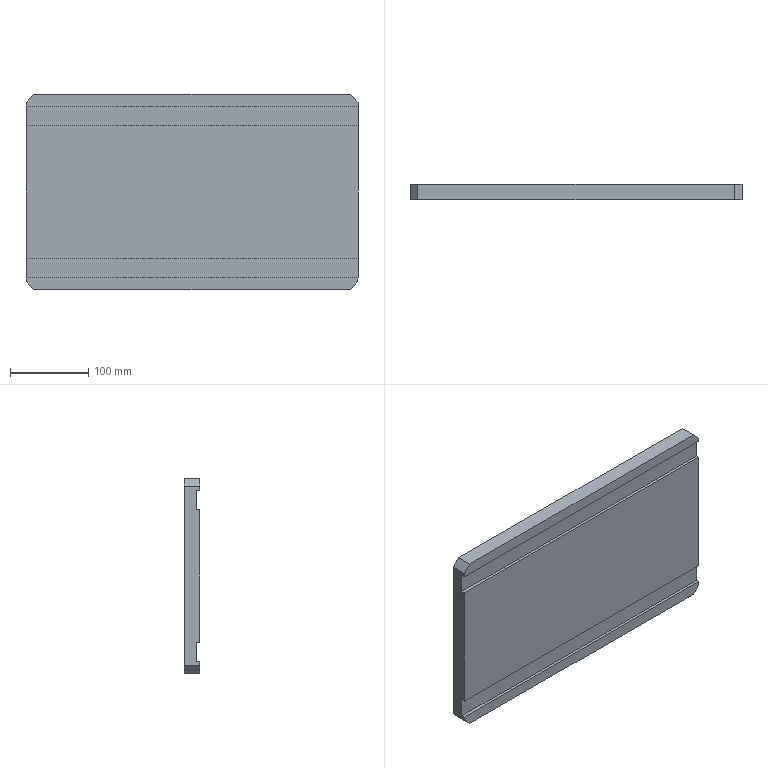Component | SolidWorks | 100-04-1 | 1 solid | 18 faces | box 425 x 20 x 250 mm | volume 2036000 mm3 | plane 18 | material 45
build123d program:
from build123d import *

# Parameters (mm, degrees)
SKETCH1_W           = 250
SKETCH1_H           = 425
BOSS_EXTRUDE1_DEPTH = 10
CHAMFER1_SIZE       = 10
SKETCH5_W           = 25
SKETCH5_H           = 425
CUT_EXTRUDE1_DEPTH  = 4


with BuildPart() as part:
    # Sketch1 → Boss-Extrude1 (new, symmetric)
    with BuildSketch(Plane(origin=(0, 0, 0), x_dir=(1, 0, 0), z_dir=(0, 1, 0))):
        Rectangle(SKETCH1_W, SKETCH1_H)
    extrude(amount=BOSS_EXTRUDE1_DEPTH, both=True)

    # Chamfer1
    chamfer1_edges = [part.edges().sort_by_distance(p)[0] for p in [
        (-125, 0, -212.5),
        (125, 0, -212.5),
        (125, 0, 212.5),
        (-125, 0, 212.5),
    ]]
    chamfer(chamfer1_edges, length=CHAMFER1_SIZE)

    # Sketch5 → Cut-Extrude1 (cut)
    with BuildSketch(Plane.XZ.offset(10)):
        with Locations((-97.5, 0)):
            Rectangle(SKETCH5_W, SKETCH5_H)
    cut_extrude1 = extrude(amount=-CUT_EXTRUDE1_DEPTH, mode=Mode.SUBTRACT)

    # Mirror1: Cut-Extrude1 across plane
    add(cut_extrude1.mirror(Plane(origin=(0, 0, 0), x_dir=(0, 0, 1), z_dir=(1, 0, 0))), mode=Mode.SUBTRACT)


solid = part.part

# Placed as in the assembly
solid = solid.moved(Location((-33.5, 990, 0), (0, 90, 0)))
STEP:
#1=COLOUR_RGB('',0.7922,0.8196,0.9333);
#2=FILL_AREA_STYLE_COLOUR('',#1);
#3=FILL_AREA_STYLE('',(#2));
#4=SURFACE_STYLE_FILL_AREA(#3);
#5=SURFACE_SIDE_STYLE('',(#4));
#6=SURFACE_STYLE_USAGE(.BOTH.,#5);
#7=PRESENTATION_STYLE_ASSIGNMENT((#6));
#8=CARTESIAN_POINT('',(7.047,38.583,3.346));
#9=VERTEX_POINT('',#8);
#10=CARTESIAN_POINT('',(-9.685,38.583,3.346));
#11=VERTEX_POINT('',#10);
#12=CARTESIAN_POINT('',(-9.685,38.583,3.346));
#13=DIRECTION('',(-1.,0.,0.));
#14=VECTOR('',#13,39.37);
#15=LINE('',#12,#14);
#16=EDGE_CURVE('',#9,#11,#15,.T.);
#17=ORIENTED_EDGE('',*,*,#16,.T.);
#18=CARTESIAN_POINT('',(-9.685,38.583,-3.346));
#19=VERTEX_POINT('',#18);
#20=CARTESIAN_POINT('',(-9.685,38.583,4.921));
#21=DIRECTION('',(0.,0.,1.));
#22=VECTOR('',#21,39.37);
#23=LINE('',#20,#22);
#24=EDGE_CURVE('',#19,#11,#23,.T.);
#25=ORIENTED_EDGE('',*,*,#24,.F.);
#26=CARTESIAN_POINT('',(7.047,38.583,-3.346));
#27=VERTEX_POINT('',#26);
#28=CARTESIAN_POINT('',(-9.685,38.583,-3.346));
#29=DIRECTION('',(-1.,0.,-0.));
#30=VECTOR('',#29,39.37);
#31=LINE('',#28,#30);
#32=EDGE_CURVE('',#27,#19,#31,.T.);
#33=ORIENTED_EDGE('',*,*,#32,.F.);
#34=CARTESIAN_POINT('',(7.047,38.583,4.921));
#35=DIRECTION('',(-0.,-0.,-1.));
#36=VECTOR('',#35,39.37);
#37=LINE('',#34,#36);
#38=EDGE_CURVE('',#9,#27,#37,.T.);
#39=ORIENTED_EDGE('',*,*,#38,.F.);
#40=EDGE_LOOP('',(#17,#25,#33,#39));
#41=FACE_OUTER_BOUND('',#40,.T.);
#42=CARTESIAN_POINT('',(-1.319,38.583,-0.));
#43=DIRECTION('',(-0.,1.,-0.));
#44=DIRECTION('',(-1.,-0.,0.));
#45=AXIS2_PLACEMENT_3D('',#42,#43,#44);
#46=PLANE('',#45);
#47=ADVANCED_FACE('',(#41),#46,.F.);
#48=CARTESIAN_POINT('',(-9.685,38.583,4.331));
#49=VERTEX_POINT('',#48);
#50=CARTESIAN_POINT('',(7.047,38.583,4.331));
#51=VERTEX_POINT('',#50);
#52=CARTESIAN_POINT('',(-9.685,38.583,4.331));
#53=DIRECTION('',(1.,-0.,-0.));
#54=VECTOR('',#53,39.37);
#55=LINE('',#52,#54);
#56=EDGE_CURVE('',#49,#51,#55,.T.);
#57=ORIENTED_EDGE('',*,*,#56,.T.);
#58=CARTESIAN_POINT('',(7.047,38.583,4.528));
#59=VERTEX_POINT('',#58);
#60=CARTESIAN_POINT('',(7.047,38.583,4.921));
#61=DIRECTION('',(-0.,-0.,-1.));
#62=VECTOR('',#61,39.37);
#63=LINE('',#60,#62);
#64=EDGE_CURVE('',#59,#51,#63,.T.);
#65=ORIENTED_EDGE('',*,*,#64,.F.);
#66=CARTESIAN_POINT('',(6.654,38.583,4.921));
#67=VERTEX_POINT('',#66);
#68=CARTESIAN_POINT('',(7.047,38.583,4.528));
#69=DIRECTION('',(-0.7071,0.,0.7071));
#70=VECTOR('',#69,39.37);
#71=LINE('',#68,#70);
#72=EDGE_CURVE('',#59,#67,#71,.T.);
#73=ORIENTED_EDGE('',*,*,#72,.T.);
#74=CARTESIAN_POINT('',(-9.291,38.583,4.921));
#75=VERTEX_POINT('',#74);
#76=CARTESIAN_POINT('',(-9.685,38.583,4.921));
#77=DIRECTION('',(1.,0.,0.));
#78=VECTOR('',#77,39.37);
#79=LINE('',#76,#78);
#80=EDGE_CURVE('',#75,#67,#79,.T.);
#81=ORIENTED_EDGE('',*,*,#80,.F.);
#82=CARTESIAN_POINT('',(-9.685,38.583,4.528));
#83=VERTEX_POINT('',#82);
#84=CARTESIAN_POINT('',(-9.291,38.583,4.921));
#85=DIRECTION('',(-0.7071,-0.,-0.7071));
#86=VECTOR('',#85,39.37);
#87=LINE('',#84,#86);
#88=EDGE_CURVE('',#75,#83,#87,.T.);
#89=ORIENTED_EDGE('',*,*,#88,.T.);
#90=CARTESIAN_POINT('',(-9.685,38.583,4.921));
#91=DIRECTION('',(0.,0.,1.));
#92=VECTOR('',#91,39.37);
#93=LINE('',#90,#92);
#94=EDGE_CURVE('',#49,#83,#93,.T.);
#95=ORIENTED_EDGE('',*,*,#94,.F.);
#96=EDGE_LOOP('',(#57,#65,#73,#81,#89,#95));
#97=FACE_OUTER_BOUND('',#96,.T.);
#98=CARTESIAN_POINT('',(-1.319,38.583,-0.));
#99=DIRECTION('',(-0.,1.,-0.));
#100=DIRECTION('',(-1.,-0.,0.));
#101=AXIS2_PLACEMENT_3D('',#98,#99,#100);
#102=PLANE('',#101);
#103=ADVANCED_FACE('',(#97),#102,.F.);
#104=CARTESIAN_POINT('',(-9.685,38.74,3.346));
#105=VERTEX_POINT('',#104);
#106=CARTESIAN_POINT('',(-9.685,38.74,3.346));
#107=DIRECTION('',(-0.,-1.,0.));
#108=VECTOR('',#107,39.37);
#109=LINE('',#106,#108);
#110=EDGE_CURVE('',#105,#11,#109,.T.);
#111=ORIENTED_EDGE('',*,*,#110,.F.);
#112=CARTESIAN_POINT('',(-9.685,38.74,4.331));
#113=VERTEX_POINT('',#112);
#114=CARTESIAN_POINT('',(-9.685,38.74,3.346));
#115=DIRECTION('',(-0.,0.,1.));
#116=VECTOR('',#115,39.37);
#117=LINE('',#114,#116);
#118=EDGE_CURVE('',#105,#113,#117,.T.);
#119=ORIENTED_EDGE('',*,*,#118,.T.);
#120=CARTESIAN_POINT('',(-9.685,38.74,4.331));
#121=DIRECTION('',(-0.,-1.,0.));
#122=VECTOR('',#121,39.37);
#123=LINE('',#120,#122);
#124=EDGE_CURVE('',#113,#49,#123,.T.);
#125=ORIENTED_EDGE('',*,*,#124,.T.);
#126=ORIENTED_EDGE('',*,*,#94,.T.);
#127=CARTESIAN_POINT('',(-9.685,39.37,4.528));
#128=VERTEX_POINT('',#127);
#129=CARTESIAN_POINT('',(-9.685,39.37,4.528));
#130=DIRECTION('',(0.,1.,-0.));
#131=VECTOR('',#130,39.37);
#132=LINE('',#129,#131);
#133=EDGE_CURVE('',#83,#128,#132,.T.);
#134=ORIENTED_EDGE('',*,*,#133,.T.);
#135=CARTESIAN_POINT('',(-9.685,39.37,-4.528));
#136=VERTEX_POINT('',#135);
#137=CARTESIAN_POINT('',(-9.685,39.37,4.921));
#138=DIRECTION('',(0.,0.,1.));
#139=VECTOR('',#138,39.37);
#140=LINE('',#137,#139);
#141=EDGE_CURVE('',#136,#128,#140,.T.);
#142=ORIENTED_EDGE('',*,*,#141,.F.);
#143=CARTESIAN_POINT('',(-9.685,38.583,-4.528));
#144=VERTEX_POINT('',#143);
#145=CARTESIAN_POINT('',(-9.685,39.37,-4.528));
#146=DIRECTION('',(-0.,-1.,0.));
#147=VECTOR('',#146,39.37);
#148=LINE('',#145,#147);
#149=EDGE_CURVE('',#136,#144,#148,.T.);
#150=ORIENTED_EDGE('',*,*,#149,.T.);
#151=CARTESIAN_POINT('',(-9.685,38.583,-4.331));
#152=VERTEX_POINT('',#151);
#153=CARTESIAN_POINT('',(-9.685,38.583,4.921));
#154=DIRECTION('',(0.,0.,1.));
#155=VECTOR('',#154,39.37);
#156=LINE('',#153,#155);
#157=EDGE_CURVE('',#144,#152,#156,.T.);
#158=ORIENTED_EDGE('',*,*,#157,.T.);
#159=CARTESIAN_POINT('',(-9.685,38.74,-4.331));
#160=VERTEX_POINT('',#159);
#161=CARTESIAN_POINT('',(-9.685,38.74,-4.331));
#162=DIRECTION('',(-0.,-1.,0.));
#163=VECTOR('',#162,39.37);
#164=LINE('',#161,#163);
#165=EDGE_CURVE('',#160,#152,#164,.T.);
#166=ORIENTED_EDGE('',*,*,#165,.F.);
#167=CARTESIAN_POINT('',(-9.685,38.74,-3.346));
#168=VERTEX_POINT('',#167);
#169=CARTESIAN_POINT('',(-9.685,38.74,-3.346));
#170=DIRECTION('',(-0.,-0.,-1.));
#171=VECTOR('',#170,39.37);
#172=LINE('',#169,#171);
#173=EDGE_CURVE('',#168,#160,#172,.T.);
#174=ORIENTED_EDGE('',*,*,#173,.F.);
#175=CARTESIAN_POINT('',(-9.685,38.74,-3.346));
#176=DIRECTION('',(-0.,-1.,0.));
#177=VECTOR('',#176,39.37);
#178=LINE('',#175,#177);
#179=EDGE_CURVE('',#168,#19,#178,.T.);
#180=ORIENTED_EDGE('',*,*,#179,.T.);
#181=ORIENTED_EDGE('',*,*,#24,.T.);
#182=EDGE_LOOP('',(#111,#119,#125,#126,#134,#142,#150,#158,#166,#174,#180,#181));
#183=FACE_OUTER_BOUND('',#182,.T.);
#184=CARTESIAN_POINT('',(-9.685,39.37,4.921));
#185=DIRECTION('',(1.,0.,-0.));
#186=DIRECTION('',(-0.,-0.,-1.));
#187=AXIS2_PLACEMENT_3D('',#184,#185,#186);
#188=PLANE('',#187);
#189=ADVANCED_FACE('',(#183),#188,.F.);
#190=CARTESIAN_POINT('',(7.047,38.74,3.346));
#191=VERTEX_POINT('',#190);
#192=CARTESIAN_POINT('',(7.047,38.74,3.346));
#193=DIRECTION('',(-0.,-1.,0.));
#194=VECTOR('',#193,39.37);
#195=LINE('',#192,#194);
#196=EDGE_CURVE('',#191,#9,#195,.T.);
#197=ORIENTED_EDGE('',*,*,#196,.T.);
#198=ORIENTED_EDGE('',*,*,#38,.T.);
#199=CARTESIAN_POINT('',(7.047,38.74,-3.346));
#200=VERTEX_POINT('',#199);
#201=CARTESIAN_POINT('',(7.047,38.74,-3.346));
#202=DIRECTION('',(-0.,-1.,0.));
#203=VECTOR('',#202,39.37);
#204=LINE('',#201,#203);
#205=EDGE_CURVE('',#200,#27,#204,.T.);
#206=ORIENTED_EDGE('',*,*,#205,.F.);
#207=CARTESIAN_POINT('',(7.047,38.74,-4.331));
#208=VERTEX_POINT('',#207);
#209=CARTESIAN_POINT('',(7.047,38.74,-3.346));
#210=DIRECTION('',(0.,0.,1.));
#211=VECTOR('',#210,39.37);
#212=LINE('',#209,#211);
#213=EDGE_CURVE('',#208,#200,#212,.T.);
#214=ORIENTED_EDGE('',*,*,#213,.F.);
#215=CARTESIAN_POINT('',(7.047,38.583,-4.331));
#216=VERTEX_POINT('',#215);
#217=CARTESIAN_POINT('',(7.047,38.74,-4.331));
#218=DIRECTION('',(-0.,-1.,0.));
#219=VECTOR('',#218,39.37);
#220=LINE('',#217,#219);
#221=EDGE_CURVE('',#208,#216,#220,.T.);
#222=ORIENTED_EDGE('',*,*,#221,.T.);
#223=CARTESIAN_POINT('',(7.047,38.583,-4.528));
#224=VERTEX_POINT('',#223);
#225=CARTESIAN_POINT('',(7.047,38.583,4.921));
#226=DIRECTION('',(-0.,-0.,-1.));
#227=VECTOR('',#226,39.37);
#228=LINE('',#225,#227);
#229=EDGE_CURVE('',#216,#224,#228,.T.);
#230=ORIENTED_EDGE('',*,*,#229,.T.);
#231=CARTESIAN_POINT('',(7.047,39.37,-4.528));
#232=VERTEX_POINT('',#231);
#233=CARTESIAN_POINT('',(7.047,39.37,-4.528));
#234=DIRECTION('',(0.,1.,-0.));
#235=VECTOR('',#234,39.37);
#236=LINE('',#233,#235);
#237=EDGE_CURVE('',#224,#232,#236,.T.);
#238=ORIENTED_EDGE('',*,*,#237,.T.);
#239=CARTESIAN_POINT('',(7.047,39.37,4.528));
#240=VERTEX_POINT('',#239);
#241=CARTESIAN_POINT('',(7.047,39.37,4.921));
#242=DIRECTION('',(-0.,-0.,-1.));
#243=VECTOR('',#242,39.37);
#244=LINE('',#241,#243);
#245=EDGE_CURVE('',#240,#232,#244,.T.);
#246=ORIENTED_EDGE('',*,*,#245,.F.);
#247=CARTESIAN_POINT('',(7.047,39.37,4.528));
#248=DIRECTION('',(-0.,-1.,0.));
#249=VECTOR('',#248,39.37);
#250=LINE('',#247,#249);
#251=EDGE_CURVE('',#240,#59,#250,.T.);
#252=ORIENTED_EDGE('',*,*,#251,.T.);
#253=ORIENTED_EDGE('',*,*,#64,.T.);
#254=CARTESIAN_POINT('',(7.047,38.74,4.331));
#255=VERTEX_POINT('',#254);
#256=CARTESIAN_POINT('',(7.047,38.74,4.331));
#257=DIRECTION('',(-0.,-1.,0.));
#258=VECTOR('',#257,39.37);
#259=LINE('',#256,#258);
#260=EDGE_CURVE('',#255,#51,#259,.T.);
#261=ORIENTED_EDGE('',*,*,#260,.F.);
#262=CARTESIAN_POINT('',(7.047,38.74,3.346));
#263=DIRECTION('',(0.,-0.,-1.));
#264=VECTOR('',#263,39.37);
#265=LINE('',#262,#264);
#266=EDGE_CURVE('',#255,#191,#265,.T.);
#267=ORIENTED_EDGE('',*,*,#266,.T.);
#268=EDGE_LOOP('',(#197,#198,#206,#214,#222,#230,#238,#246,#252,#253,#261,#267));
#269=FACE_OUTER_BOUND('',#268,.T.);
#270=CARTESIAN_POINT('',(7.047,39.37,4.921));
#271=DIRECTION('',(-1.,-0.,0.));
#272=DIRECTION('',(0.,0.,1.));
#273=AXIS2_PLACEMENT_3D('',#270,#271,#272);
#274=PLANE('',#273);
#275=ADVANCED_FACE('',(#269),#274,.F.);
#276=CARTESIAN_POINT('',(6.654,38.583,-4.921));
#277=VERTEX_POINT('',#276);
#278=CARTESIAN_POINT('',(-9.291,38.583,-4.921));
#279=VERTEX_POINT('',#278);
#280=CARTESIAN_POINT('',(-9.685,38.583,-4.921));
#281=DIRECTION('',(-1.,-0.,0.));
#282=VECTOR('',#281,39.37);
#283=LINE('',#280,#282);
#284=EDGE_CURVE('',#277,#279,#283,.T.);
#285=ORIENTED_EDGE('',*,*,#284,.T.);
#286=CARTESIAN_POINT('',(-9.291,39.37,-4.921));
#287=VERTEX_POINT('',#286);
#288=CARTESIAN_POINT('',(-9.291,39.37,-4.921));
#289=DIRECTION('',(0.,1.,-0.));
#290=VECTOR('',#289,39.37);
#291=LINE('',#288,#290);
#292=EDGE_CURVE('',#279,#287,#291,.T.);
#293=ORIENTED_EDGE('',*,*,#292,.T.);
#294=CARTESIAN_POINT('',(6.654,39.37,-4.921));
#295=VERTEX_POINT('',#294);
#296=CARTESIAN_POINT('',(-9.685,39.37,-4.921));
#297=DIRECTION('',(-1.,-0.,0.));
#298=VECTOR('',#297,39.37);
#299=LINE('',#296,#298);
#300=EDGE_CURVE('',#295,#287,#299,.T.);
#301=ORIENTED_EDGE('',*,*,#300,.F.);
#302=CARTESIAN_POINT('',(6.654,39.37,-4.921));
#303=DIRECTION('',(-0.,-1.,0.));
#304=VECTOR('',#303,39.37);
#305=LINE('',#302,#304);
#306=EDGE_CURVE('',#295,#277,#305,.T.);
#307=ORIENTED_EDGE('',*,*,#306,.T.);
#308=EDGE_LOOP('',(#285,#293,#301,#307));
#309=FACE_OUTER_BOUND('',#308,.T.);
#310=CARTESIAN_POINT('',(-9.685,39.37,-4.921));
#311=DIRECTION('',(-0.,0.,1.));
#312=DIRECTION('',(1.,0.,0.));
#313=AXIS2_PLACEMENT_3D('',#310,#311,#312);
#314=PLANE('',#313);
#315=ADVANCED_FACE('',(#309),#314,.F.);
#316=CARTESIAN_POINT('',(-9.291,39.37,4.921));
#317=VERTEX_POINT('',#316);
#318=CARTESIAN_POINT('',(6.654,39.37,4.921));
#319=VERTEX_POINT('',#318);
#320=CARTESIAN_POINT('',(-9.685,39.37,4.921));
#321=DIRECTION('',(1.,0.,0.));
#322=VECTOR('',#321,39.37);
#323=LINE('',#320,#322);
#324=EDGE_CURVE('',#317,#319,#323,.T.);
#325=ORIENTED_EDGE('',*,*,#324,.F.);
#326=CARTESIAN_POINT('',(-9.291,39.37,4.921));
#327=DIRECTION('',(-0.,-1.,0.));
#328=VECTOR('',#327,39.37);
#329=LINE('',#326,#328);
#330=EDGE_CURVE('',#317,#75,#329,.T.);
#331=ORIENTED_EDGE('',*,*,#330,.T.);
#332=ORIENTED_EDGE('',*,*,#80,.T.);
#333=CARTESIAN_POINT('',(6.654,39.37,4.921));
#334=DIRECTION('',(0.,1.,-0.));
#335=VECTOR('',#334,39.37);
#336=LINE('',#333,#335);
#337=EDGE_CURVE('',#67,#319,#336,.T.);
#338=ORIENTED_EDGE('',*,*,#337,.T.);
#339=EDGE_LOOP('',(#325,#331,#332,#338));
#340=FACE_OUTER_BOUND('',#339,.T.);
#341=CARTESIAN_POINT('',(-9.685,39.37,4.921));
#342=DIRECTION('',(0.,-0.,-1.));
#343=DIRECTION('',(-1.,-0.,0.));
#344=AXIS2_PLACEMENT_3D('',#341,#342,#343);
#345=PLANE('',#344);
#346=ADVANCED_FACE('',(#340),#345,.F.);
#347=ORIENTED_EDGE('',*,*,#300,.T.);
#348=CARTESIAN_POINT('',(-7.766,39.37,-6.447));
#349=DIRECTION('',(-0.7071,0.,0.7071));
#350=VECTOR('',#349,39.37);
#351=LINE('',#348,#350);
#352=EDGE_CURVE('',#287,#136,#351,.T.);
#353=ORIENTED_EDGE('',*,*,#352,.T.);
#354=ORIENTED_EDGE('',*,*,#141,.T.);
#355=CARTESIAN_POINT('',(-7.766,39.37,6.447));
#356=DIRECTION('',(0.7071,0.,0.7071));
#357=VECTOR('',#356,39.37);
#358=LINE('',#355,#357);
#359=EDGE_CURVE('',#128,#317,#358,.T.);
#360=ORIENTED_EDGE('',*,*,#359,.T.);
#361=ORIENTED_EDGE('',*,*,#324,.T.);
#362=CARTESIAN_POINT('',(5.128,39.37,6.447));
#363=DIRECTION('',(0.7071,-0.,-0.7071));
#364=VECTOR('',#363,39.37);
#365=LINE('',#362,#364);
#366=EDGE_CURVE('',#319,#240,#365,.T.);
#367=ORIENTED_EDGE('',*,*,#366,.T.);
#368=ORIENTED_EDGE('',*,*,#245,.T.);
#369=CARTESIAN_POINT('',(5.128,39.37,-6.447));
#370=DIRECTION('',(-0.7071,-0.,-0.7071));
#371=VECTOR('',#370,39.37);
#372=LINE('',#369,#371);
#373=EDGE_CURVE('',#232,#295,#372,.T.);
#374=ORIENTED_EDGE('',*,*,#373,.T.);
#375=EDGE_LOOP('',(#347,#353,#354,#360,#361,#367,#368,#374));
#376=FACE_OUTER_BOUND('',#375,.T.);
#377=CARTESIAN_POINT('',(-1.319,39.37,-0.));
#378=DIRECTION('',(-0.,1.,-0.));
#379=DIRECTION('',(-1.,-0.,0.));
#380=AXIS2_PLACEMENT_3D('',#377,#378,#379);
#381=PLANE('',#380);
#382=ADVANCED_FACE('',(#376),#381,.T.);
#383=ORIENTED_EDGE('',*,*,#229,.F.);
#384=CARTESIAN_POINT('',(-9.685,38.583,-4.331));
#385=DIRECTION('',(1.,-0.,0.));
#386=VECTOR('',#385,39.37);
#387=LINE('',#384,#386);
#388=EDGE_CURVE('',#152,#216,#387,.T.);
#389=ORIENTED_EDGE('',*,*,#388,.F.);
#390=ORIENTED_EDGE('',*,*,#157,.F.);
#391=CARTESIAN_POINT('',(-9.685,38.583,-4.528));
#392=DIRECTION('',(0.7071,-0.,-0.7071));
#393=VECTOR('',#392,39.37);
#394=LINE('',#391,#393);
#395=EDGE_CURVE('',#144,#279,#394,.T.);
#396=ORIENTED_EDGE('',*,*,#395,.T.);
#397=ORIENTED_EDGE('',*,*,#284,.F.);
#398=CARTESIAN_POINT('',(6.654,38.583,-4.921));
#399=DIRECTION('',(0.7071,0.,0.7071));
#400=VECTOR('',#399,39.37);
#401=LINE('',#398,#400);
#402=EDGE_CURVE('',#277,#224,#401,.T.);
#403=ORIENTED_EDGE('',*,*,#402,.T.);
#404=EDGE_LOOP('',(#383,#389,#390,#396,#397,#403));
#405=FACE_OUTER_BOUND('',#404,.T.);
#406=CARTESIAN_POINT('',(-1.319,38.583,-0.));
#407=DIRECTION('',(-0.,1.,-0.));
#408=DIRECTION('',(-1.,-0.,0.));
#409=AXIS2_PLACEMENT_3D('',#406,#407,#408);
#410=PLANE('',#409);
#411=ADVANCED_FACE('',(#405),#410,.F.);
#412=ORIENTED_EDGE('',*,*,#352,.F.);
#413=ORIENTED_EDGE('',*,*,#292,.F.);
#414=ORIENTED_EDGE('',*,*,#395,.F.);
#415=ORIENTED_EDGE('',*,*,#149,.F.);
#416=EDGE_LOOP('',(#412,#413,#414,#415));
#417=FACE_OUTER_BOUND('',#416,.T.);
#418=CARTESIAN_POINT('',(-9.685,39.37,-4.528));
#419=DIRECTION('',(0.7071,0.,0.7071));
#420=DIRECTION('',(-0.,-1.,0.));
#421=AXIS2_PLACEMENT_3D('',#418,#419,#420);
#422=PLANE('',#421);
#423=ADVANCED_FACE('',(#417),#422,.F.);
#424=ORIENTED_EDGE('',*,*,#359,.F.);
#425=ORIENTED_EDGE('',*,*,#133,.F.);
#426=ORIENTED_EDGE('',*,*,#88,.F.);
#427=ORIENTED_EDGE('',*,*,#330,.F.);
#428=EDGE_LOOP('',(#424,#425,#426,#427));
#429=FACE_OUTER_BOUND('',#428,.T.);
#430=CARTESIAN_POINT('',(-9.291,39.37,4.921));
#431=DIRECTION('',(0.7071,-0.,-0.7071));
#432=DIRECTION('',(-0.,-1.,0.));
#433=AXIS2_PLACEMENT_3D('',#430,#431,#432);
#434=PLANE('',#433);
#435=ADVANCED_FACE('',(#429),#434,.F.);
#436=ORIENTED_EDGE('',*,*,#366,.F.);
#437=ORIENTED_EDGE('',*,*,#337,.F.);
#438=ORIENTED_EDGE('',*,*,#72,.F.);
#439=ORIENTED_EDGE('',*,*,#251,.F.);
#440=EDGE_LOOP('',(#436,#437,#438,#439));
#441=FACE_OUTER_BOUND('',#440,.T.);
#442=CARTESIAN_POINT('',(7.047,39.37,4.528));
#443=DIRECTION('',(-0.7071,-0.,-0.7071));
#444=DIRECTION('',(-0.,-1.,0.));
#445=AXIS2_PLACEMENT_3D('',#442,#443,#444);
#446=PLANE('',#445);
#447=ADVANCED_FACE('',(#441),#446,.F.);
#448=ORIENTED_EDGE('',*,*,#373,.F.);
#449=ORIENTED_EDGE('',*,*,#237,.F.);
#450=ORIENTED_EDGE('',*,*,#402,.F.);
#451=ORIENTED_EDGE('',*,*,#306,.F.);
#452=EDGE_LOOP('',(#448,#449,#450,#451));
#453=FACE_OUTER_BOUND('',#452,.T.);
#454=CARTESIAN_POINT('',(6.654,39.37,-4.921));
#455=DIRECTION('',(-0.7071,0.,0.7071));
#456=DIRECTION('',(-0.,-1.,0.));
#457=AXIS2_PLACEMENT_3D('',#454,#455,#456);
#458=PLANE('',#457);
#459=ADVANCED_FACE('',(#453),#458,.F.);
#460=ORIENTED_EDGE('',*,*,#32,.T.);
#461=ORIENTED_EDGE('',*,*,#179,.F.);
#462=CARTESIAN_POINT('',(-9.685,38.74,-3.346));
#463=DIRECTION('',(-1.,0.,-0.));
#464=VECTOR('',#463,39.37);
#465=LINE('',#462,#464);
#466=EDGE_CURVE('',#200,#168,#465,.T.);
#467=ORIENTED_EDGE('',*,*,#466,.F.);
#468=ORIENTED_EDGE('',*,*,#205,.T.);
#469=EDGE_LOOP('',(#460,#461,#467,#468));
#470=FACE_OUTER_BOUND('',#469,.T.);
#471=CARTESIAN_POINT('',(-9.685,38.74,-3.346));
#472=DIRECTION('',(-0.,0.,1.));
#473=DIRECTION('',(1.,0.,0.));
#474=AXIS2_PLACEMENT_3D('',#471,#472,#473);
#475=PLANE('',#474);
#476=ADVANCED_FACE('',(#470),#475,.F.);
#477=ORIENTED_EDGE('',*,*,#388,.T.);
#478=ORIENTED_EDGE('',*,*,#221,.F.);
#479=CARTESIAN_POINT('',(-9.685,38.74,-4.331));
#480=DIRECTION('',(1.,-0.,0.));
#481=VECTOR('',#480,39.37);
#482=LINE('',#479,#481);
#483=EDGE_CURVE('',#160,#208,#482,.T.);
#484=ORIENTED_EDGE('',*,*,#483,.F.);
#485=ORIENTED_EDGE('',*,*,#165,.T.);
#486=EDGE_LOOP('',(#477,#478,#484,#485));
#487=FACE_OUTER_BOUND('',#486,.T.);
#488=CARTESIAN_POINT('',(-9.685,38.74,-4.331));
#489=DIRECTION('',(0.,-0.,-1.));
#490=DIRECTION('',(-1.,-0.,-0.));
#491=AXIS2_PLACEMENT_3D('',#488,#489,#490);
#492=PLANE('',#491);
#493=ADVANCED_FACE('',(#487),#492,.F.);
#494=ORIENTED_EDGE('',*,*,#466,.T.);
#495=ORIENTED_EDGE('',*,*,#173,.T.);
#496=ORIENTED_EDGE('',*,*,#483,.T.);
#497=ORIENTED_EDGE('',*,*,#213,.T.);
#498=EDGE_LOOP('',(#494,#495,#496,#497));
#499=FACE_OUTER_BOUND('',#498,.T.);
#500=CARTESIAN_POINT('',(-1.319,38.74,-0.));
#501=DIRECTION('',(0.,1.,-0.));
#502=DIRECTION('',(-1.,0.,-0.));
#503=AXIS2_PLACEMENT_3D('',#500,#501,#502);
#504=PLANE('',#503);
#505=ADVANCED_FACE('',(#499),#504,.F.);
#506=ORIENTED_EDGE('',*,*,#16,.F.);
#507=ORIENTED_EDGE('',*,*,#196,.F.);
#508=CARTESIAN_POINT('',(-9.685,38.74,3.346));
#509=DIRECTION('',(-1.,0.,0.));
#510=VECTOR('',#509,39.37);
#511=LINE('',#508,#510);
#512=EDGE_CURVE('',#191,#105,#511,.T.);
#513=ORIENTED_EDGE('',*,*,#512,.T.);
#514=ORIENTED_EDGE('',*,*,#110,.T.);
#515=EDGE_LOOP('',(#506,#507,#513,#514));
#516=FACE_OUTER_BOUND('',#515,.T.);
#517=CARTESIAN_POINT('',(-9.685,38.74,3.346));
#518=DIRECTION('',(0.,0.,1.));
#519=DIRECTION('',(1.,0.,-0.));
#520=AXIS2_PLACEMENT_3D('',#517,#518,#519);
#521=PLANE('',#520);
#522=ADVANCED_FACE('',(#516),#521,.T.);
#523=ORIENTED_EDGE('',*,*,#56,.F.);
#524=ORIENTED_EDGE('',*,*,#124,.F.);
#525=CARTESIAN_POINT('',(-9.685,38.74,4.331));
#526=DIRECTION('',(1.,-0.,-0.));
#527=VECTOR('',#526,39.37);
#528=LINE('',#525,#527);
#529=EDGE_CURVE('',#113,#255,#528,.T.);
#530=ORIENTED_EDGE('',*,*,#529,.T.);
#531=ORIENTED_EDGE('',*,*,#260,.T.);
#532=EDGE_LOOP('',(#523,#524,#530,#531));
#533=FACE_OUTER_BOUND('',#532,.T.);
#534=CARTESIAN_POINT('',(-9.685,38.74,4.331));
#535=DIRECTION('',(-0.,-0.,-1.));
#536=DIRECTION('',(-1.,-0.,0.));
#537=AXIS2_PLACEMENT_3D('',#534,#535,#536);
#538=PLANE('',#537);
#539=ADVANCED_FACE('',(#533),#538,.T.);
#540=ORIENTED_EDGE('',*,*,#512,.F.);
#541=ORIENTED_EDGE('',*,*,#266,.F.);
#542=ORIENTED_EDGE('',*,*,#529,.F.);
#543=ORIENTED_EDGE('',*,*,#118,.F.);
#544=EDGE_LOOP('',(#540,#541,#542,#543));
#545=FACE_OUTER_BOUND('',#544,.T.);
#546=CARTESIAN_POINT('',(-1.319,38.74,-0.));
#547=DIRECTION('',(0.,1.,-0.));
#548=DIRECTION('',(-1.,0.,-0.));
#549=AXIS2_PLACEMENT_3D('',#546,#547,#548);
#550=PLANE('',#549);
#551=ADVANCED_FACE('',(#545),#550,.F.);
#552=CLOSED_SHELL('',(#47,#103,#189,#275,#315,#346,#382,#411,#423,#435,#447,#459,#476,#493,#505,#522,#539,#551));
#553=MANIFOLD_SOLID_BREP('',#552);
#554=STYLED_ITEM('',(#7),#553);
#555=PRESENTATION_LAYER_ASSIGNMENT('','',(#554));
#556=CARTESIAN_POINT('',(0.,0.,0.));
#557=DIRECTION('',(0.,0.,1.));
#558=DIRECTION('',(1.,0.,0.));
#559=AXIS2_PLACEMENT_3D('',#556,#557,#558);
#560=(LENGTH_UNIT()NAMED_UNIT(*)SI_UNIT($,.METRE.));
#561=LENGTH_MEASURE_WITH_UNIT(LENGTH_MEASURE(0.0254),#560);
#562=DIMENSIONAL_EXPONENTS(1.,0.,0.,0.,0.,0.,0.);
#563=(CONVERSION_BASED_UNIT('',#561)LENGTH_UNIT()NAMED_UNIT(#562));
#564=UNCERTAINTY_MEASURE_WITH_UNIT(LENGTH_MEASURE(0.00001),#563,'','');
#565=(NAMED_UNIT(*)PLANE_ANGLE_UNIT()SI_UNIT($,.RADIAN.));
#566=(NAMED_UNIT(*)SI_UNIT($,.STERADIAN.)SOLID_ANGLE_UNIT());
#567=(GEOMETRIC_REPRESENTATION_CONTEXT(3)GLOBAL_UNCERTAINTY_ASSIGNED_CONTEXT((#564))GLOBAL_UNIT_ASSIGNED_CONTEXT((#563,#565,#566))REPRESENTATION_CONTEXT('',''));
#568=ADVANCED_BREP_SHAPE_REPRESENTATION('',(#553,#559),#567);
#569=(LENGTH_UNIT()NAMED_UNIT(*)SI_UNIT($,.METRE.));
#570=LENGTH_MEASURE_WITH_UNIT(LENGTH_MEASURE(0.0254),#569);
#571=DIMENSIONAL_EXPONENTS(1.,0.,0.,0.,0.,0.,0.);
#572=(CONVERSION_BASED_UNIT('',#570)LENGTH_UNIT()NAMED_UNIT(#571));
#573=UNCERTAINTY_MEASURE_WITH_UNIT(LENGTH_MEASURE(0.00001),#572,'','');
#574=(NAMED_UNIT(*)PLANE_ANGLE_UNIT()SI_UNIT($,.RADIAN.));
#575=(NAMED_UNIT(*)SI_UNIT($,.STERADIAN.)SOLID_ANGLE_UNIT());
#576=(GEOMETRIC_REPRESENTATION_CONTEXT(3)GLOBAL_UNCERTAINTY_ASSIGNED_CONTEXT((#573))GLOBAL_UNIT_ASSIGNED_CONTEXT((#572,#574,#575))REPRESENTATION_CONTEXT('',''));
#577=MECHANICAL_DESIGN_GEOMETRIC_PRESENTATION_REPRESENTATION('',(#554),#576);